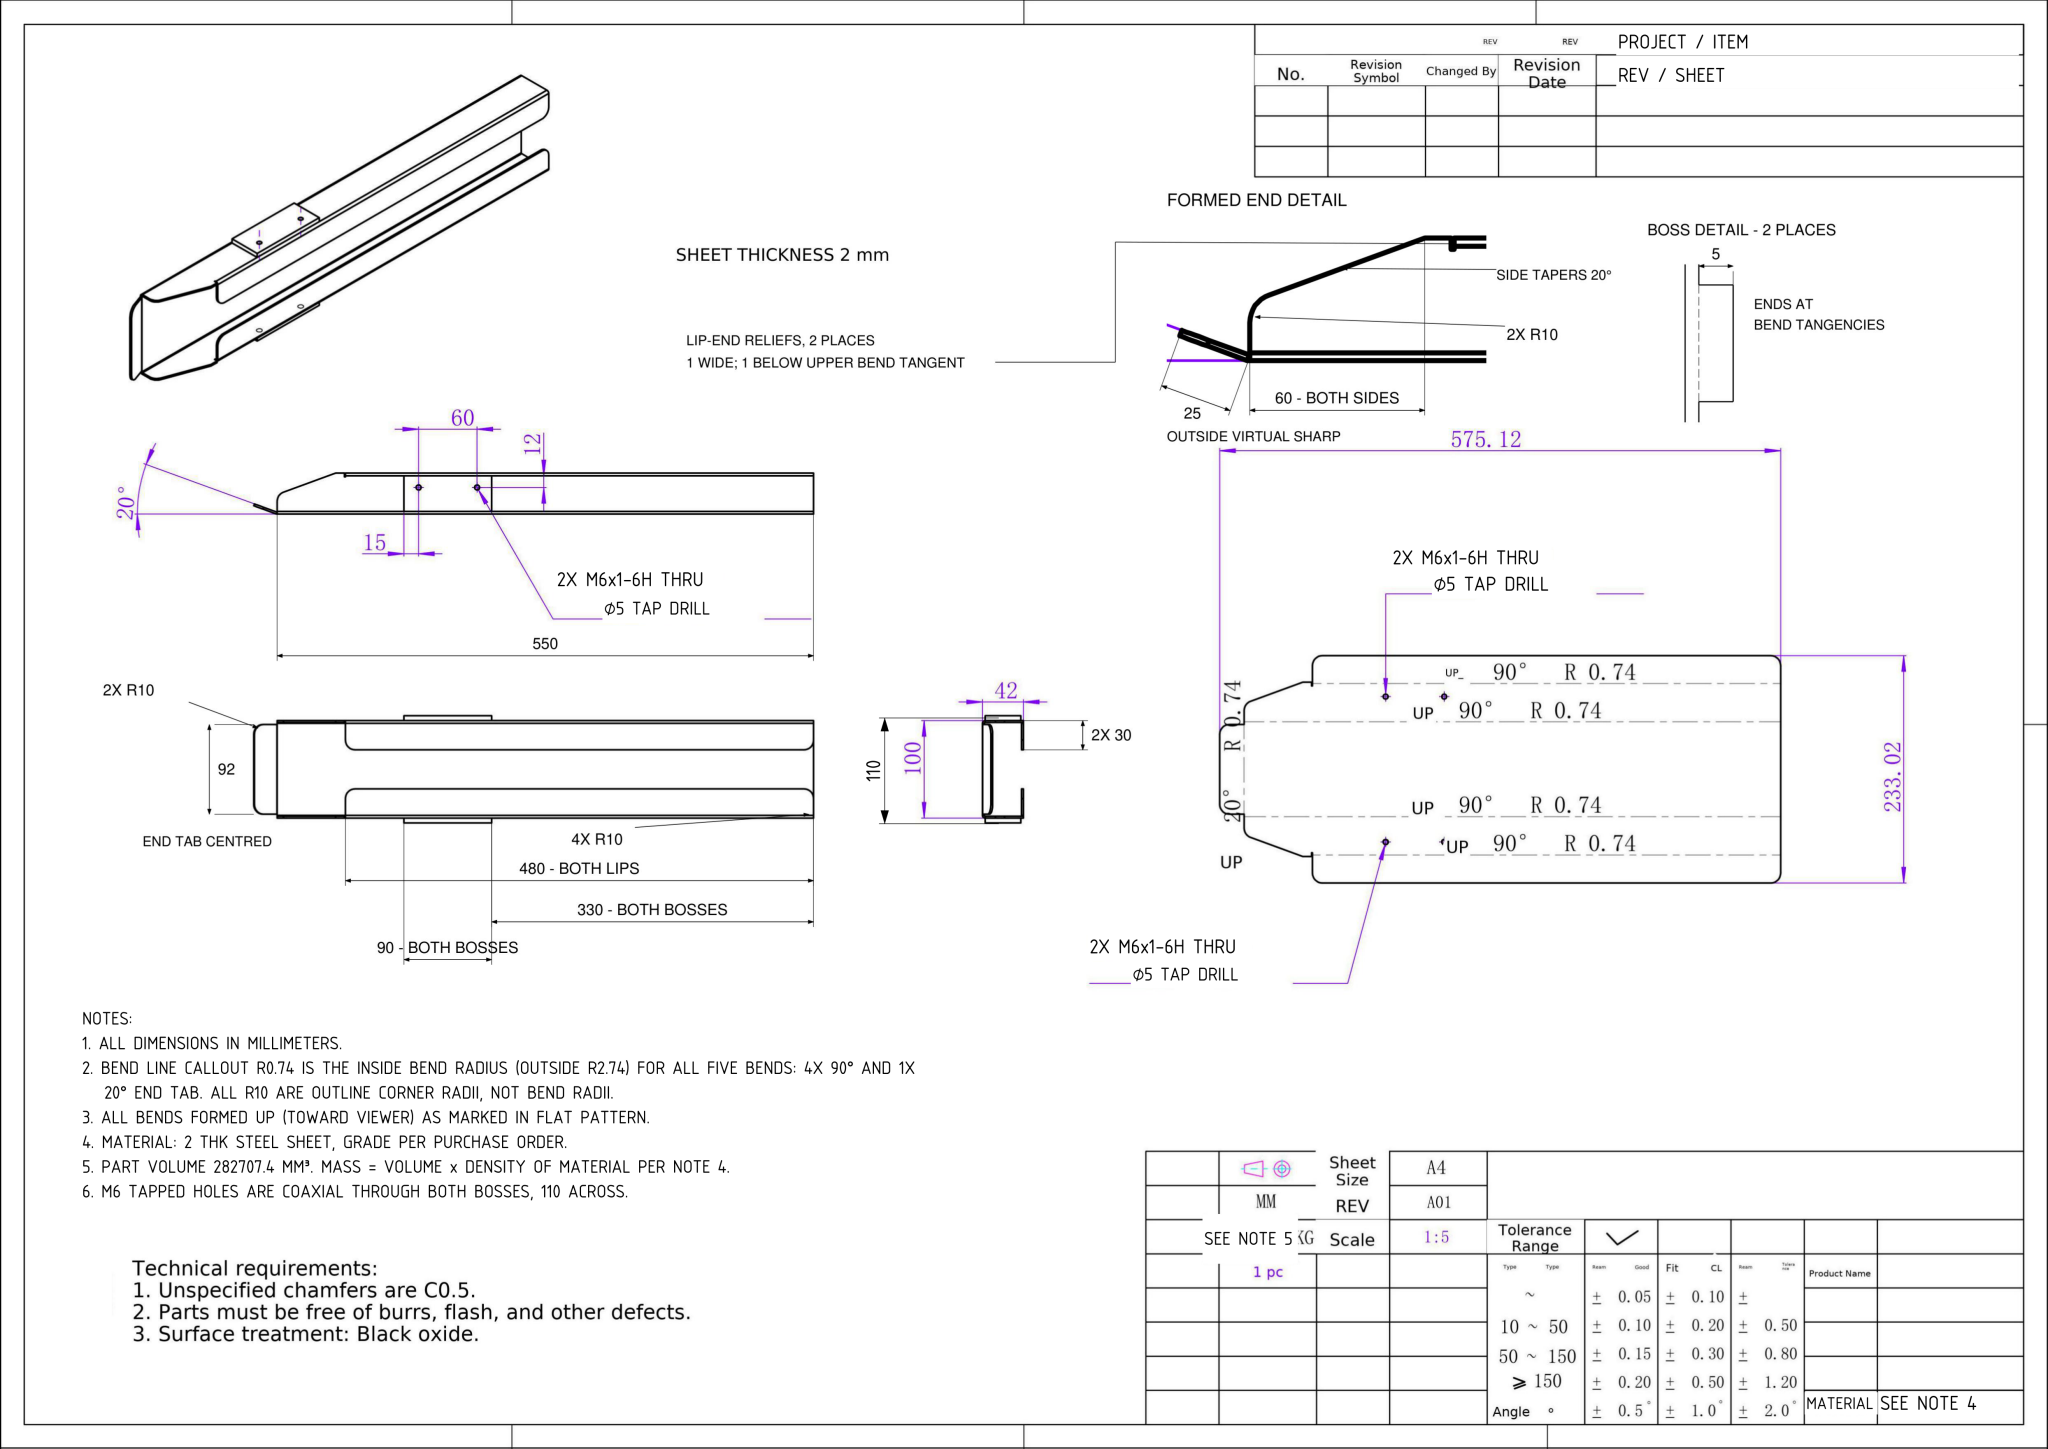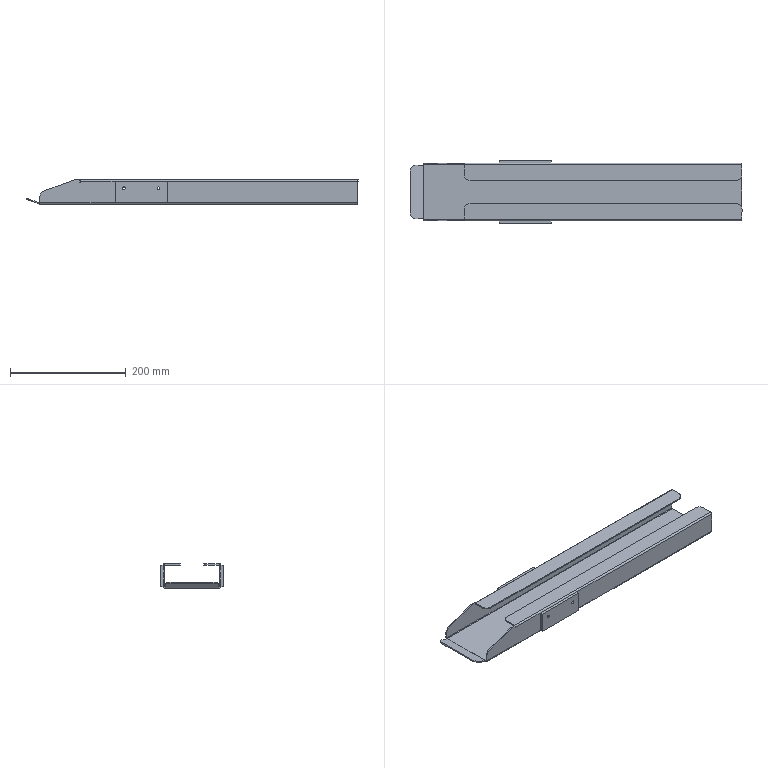Part | NX | mm | Hooked End Channel Bracket | 1 solid | 86 faces | box 573.97 x 110 x 42 mm | volume 282707 mm3 | plane 60 | cylinder 26 | commonest cylinder face diameters 5 x8 20 x8 5.473 x5 1.473 x5